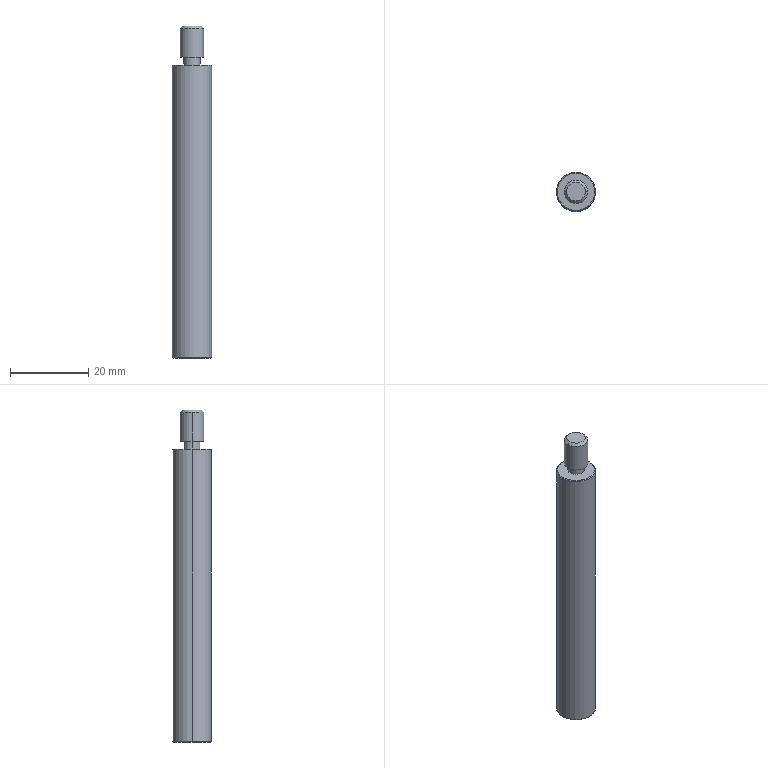Component | SolidWorks | Q1-A12-S21-Q1A.SLDASQ-1_Q1-VAFD10-75-F10-Q6-N5-1 | 1 solid | 22 faces | box 10 x 10 x 85 mm | volume 5928 mm3 | cone 10 | cylinder 8 | plane 4 | commonest cylinder face diameters 4.134 x2 6 x2 4.2 x2 10 x2
build123d program:
from build123d import *

# Parameters (mm, degrees)
SKETCH2_W = 2
SKETCH2_H = 10


with BuildPart() as part:
    # Sketch1 → Revolve1 (revolve)
    with BuildSketch(Plane.XY, mode=Mode.PRIVATE) as revolve1_sk:
        Polygon((-10, 0), (-10, 2.386), (-9.386, 3), (0, 3), (0, 4.8), (0.2, 5), (74.8, 5), (75, 4.8), (75, 0), align=None)
    revolve(revolve1_sk.sketch.rotate(Axis((75, 0, 0), (-1, 0, 0)), 270), axis=Axis((75, 0, 0), (-1, 0, 0)))

    # Sketch2 → Cut-Revolve1 (revolve, cut)
    with BuildSketch(Plane.XY, mode=Mode.PRIVATE) as cut_revolve1_sk:
        with Locations((-1, 7.1)):
            Rectangle(SKETCH2_W, SKETCH2_H)
    revolve(cut_revolve1_sk.sketch.rotate(Axis((85, 0, 0), (-1, 0, 0)), 270), axis=Axis((85, 0, 0), (-1, 0, 0)), mode=Mode.SUBTRACT)

    # Sketch3 → Cut-Revolve2 (revolve, cut)
    with BuildSketch(Plane.XY, mode=Mode.PRIVATE) as cut_revolve2_sk:
        Polygon((58.5, 0), (59.693, 2.067), (74.567, 2.067), (75, 2.5), (75, 0), align=None)
    revolve(cut_revolve2_sk.sketch.rotate(Axis((75, 0, 0), (-1, 0, 0)), 270), axis=Axis((75, 0, 0), (-1, 0, 0)), mode=Mode.SUBTRACT)


solid = part.part

# Placed as in the assembly
solid = solid.moved(Location((24.749, 24.749, -162.5), (0, 90, 0)))
STEP:
#1=COLOUR_RGB('',0.7922,0.8196,0.9333);
#2=FILL_AREA_STYLE_COLOUR('',#1);
#3=FILL_AREA_STYLE('',(#2));
#4=SURFACE_STYLE_FILL_AREA(#3);
#5=SURFACE_SIDE_STYLE('',(#4));
#6=SURFACE_STYLE_USAGE(.BOTH.,#5);
#7=PRESENTATION_STYLE_ASSIGNMENT((#6));
#8=CARTESIAN_POINT('',(0.9744,0.9744,-8.701));
#9=VERTEX_POINT('',#8);
#10=CARTESIAN_POINT('',(0.893,0.9744,-8.748));
#11=VERTEX_POINT('',#10);
#12=CARTESIAN_POINT('',(0.893,0.9744,-8.748));
#13=DIRECTION('',(-0.866,0.,-0.5));
#14=VECTOR('',#13,39.37);
#15=LINE('',#12,#14);
#16=EDGE_CURVE('',#9,#11,#15,.T.);
#17=ORIENTED_EDGE('',*,*,#16,.F.);
#18=CARTESIAN_POINT('',(1.056,0.9744,-8.748));
#19=VERTEX_POINT('',#18);
#20=CARTESIAN_POINT('',(1.056,0.9744,-8.748));
#21=DIRECTION('',(0.866,0.,-0.5));
#22=VECTOR('',#21,39.37);
#23=LINE('',#20,#22);
#24=EDGE_CURVE('',#9,#19,#23,.T.);
#25=ORIENTED_EDGE('',*,*,#24,.T.);
#26=CARTESIAN_POINT('',(0.9744,0.9744,-8.748));
#27=DIRECTION('',(0.,-0.,1.));
#28=DIRECTION('',(1.,0.,0.));
#29=AXIS2_PLACEMENT_3D('',#26,#27,#28);
#30=CIRCLE('',#29,0.08138);
#31=EDGE_CURVE('',#11,#19,#30,.T.);
#32=ORIENTED_EDGE('',*,*,#31,.F.);
#33=EDGE_LOOP('',(#17,#25,#32));
#34=FACE_OUTER_BOUND('',#33,.T.);
#35=CARTESIAN_POINT('',(0.9744,0.9744,-8.748));
#36=DIRECTION('',(-0.,0.,-1.));
#37=DIRECTION('',(-1.,0.,0.));
#38=AXIS2_PLACEMENT_3D('',#35,#36,#37);
#39=CONICAL_SURFACE('',#38,0.08138,1.047);
#40=ADVANCED_FACE('',(#34),#39,.F.);
#41=CARTESIAN_POINT('',(0.893,0.9744,-9.333));
#42=VERTEX_POINT('',#41);
#43=CARTESIAN_POINT('',(1.056,0.9744,-9.333));
#44=VERTEX_POINT('',#43);
#45=CARTESIAN_POINT('',(0.9744,0.9744,-9.333));
#46=DIRECTION('',(0.,-0.,1.));
#47=DIRECTION('',(1.,0.,0.));
#48=AXIS2_PLACEMENT_3D('',#45,#46,#47);
#49=CIRCLE('',#48,0.08138);
#50=EDGE_CURVE('',#42,#44,#49,.T.);
#51=ORIENTED_EDGE('',*,*,#50,.F.);
#52=CARTESIAN_POINT('',(0.893,0.9744,-9.35));
#53=DIRECTION('',(0.,-0.,1.));
#54=VECTOR('',#53,39.37);
#55=LINE('',#52,#54);
#56=EDGE_CURVE('',#42,#11,#55,.T.);
#57=ORIENTED_EDGE('',*,*,#56,.T.);
#58=ORIENTED_EDGE('',*,*,#31,.T.);
#59=CARTESIAN_POINT('',(1.056,0.9744,-9.35));
#60=DIRECTION('',(0.,-0.,1.));
#61=VECTOR('',#60,39.37);
#62=LINE('',#59,#61);
#63=EDGE_CURVE('',#44,#19,#62,.T.);
#64=ORIENTED_EDGE('',*,*,#63,.F.);
#65=EDGE_LOOP('',(#51,#57,#58,#64));
#66=FACE_OUTER_BOUND('',#65,.T.);
#67=CARTESIAN_POINT('',(0.9744,0.9744,-9.35));
#68=DIRECTION('',(0.,-0.,1.));
#69=DIRECTION('',(1.,0.,0.));
#70=AXIS2_PLACEMENT_3D('',#67,#68,#69);
#71=CYLINDRICAL_SURFACE('',#70,0.08138);
#72=ADVANCED_FACE('',(#66),#71,.F.);
#73=ORIENTED_EDGE('',*,*,#50,.T.);
#74=CARTESIAN_POINT('',(1.073,0.9744,-9.35));
#75=VERTEX_POINT('',#74);
#76=CARTESIAN_POINT('',(1.073,0.9744,-9.35));
#77=DIRECTION('',(0.7071,0.,-0.7071));
#78=VECTOR('',#77,39.37);
#79=LINE('',#76,#78);
#80=EDGE_CURVE('',#44,#75,#79,.T.);
#81=ORIENTED_EDGE('',*,*,#80,.T.);
#82=CARTESIAN_POINT('',(0.8759,0.9744,-9.35));
#83=VERTEX_POINT('',#82);
#84=CARTESIAN_POINT('',(0.9744,0.9744,-9.35));
#85=DIRECTION('',(0.,-0.,1.));
#86=DIRECTION('',(1.,0.,0.));
#87=AXIS2_PLACEMENT_3D('',#84,#85,#86);
#88=CIRCLE('',#87,0.09843);
#89=EDGE_CURVE('',#83,#75,#88,.T.);
#90=ORIENTED_EDGE('',*,*,#89,.F.);
#91=CARTESIAN_POINT('',(0.8759,0.9744,-9.35));
#92=DIRECTION('',(-0.7071,0.,-0.7071));
#93=VECTOR('',#92,39.37);
#94=LINE('',#91,#93);
#95=EDGE_CURVE('',#42,#83,#94,.T.);
#96=ORIENTED_EDGE('',*,*,#95,.F.);
#97=EDGE_LOOP('',(#73,#81,#90,#96));
#98=FACE_OUTER_BOUND('',#97,.T.);
#99=CARTESIAN_POINT('',(0.9744,0.9744,-9.35));
#100=DIRECTION('',(-0.,0.,-1.));
#101=DIRECTION('',(-1.,0.,0.));
#102=AXIS2_PLACEMENT_3D('',#99,#100,#101);
#103=CONICAL_SURFACE('',#102,0.09843,0.7854);
#104=ADVANCED_FACE('',(#98),#103,.F.);
#105=CARTESIAN_POINT('',(0.8562,0.9744,-6.319));
#106=VERTEX_POINT('',#105);
#107=CARTESIAN_POINT('',(1.092,0.9744,-6.319));
#108=VERTEX_POINT('',#107);
#109=CARTESIAN_POINT('',(0.9744,0.9744,-6.319));
#110=DIRECTION('',(-0.,0.,-1.));
#111=DIRECTION('',(-1.,0.,0.));
#112=AXIS2_PLACEMENT_3D('',#109,#110,#111);
#113=CIRCLE('',#112,0.1181);
#114=EDGE_CURVE('',#106,#108,#113,.T.);
#115=ORIENTED_EDGE('',*,*,#114,.F.);
#116=CARTESIAN_POINT('',(0.8562,0.9744,-6.028));
#117=VERTEX_POINT('',#116);
#118=CARTESIAN_POINT('',(0.8562,0.9744,-9.35));
#119=DIRECTION('',(0.,-0.,1.));
#120=VECTOR('',#119,39.37);
#121=LINE('',#118,#120);
#122=EDGE_CURVE('',#106,#117,#121,.T.);
#123=ORIENTED_EDGE('',*,*,#122,.T.);
#124=CARTESIAN_POINT('',(1.092,0.9744,-6.028));
#125=VERTEX_POINT('',#124);
#126=CARTESIAN_POINT('',(0.9744,0.9744,-6.028));
#127=DIRECTION('',(0.,-0.,1.));
#128=DIRECTION('',(1.,0.,0.));
#129=AXIS2_PLACEMENT_3D('',#126,#127,#128);
#130=CIRCLE('',#129,0.1181);
#131=EDGE_CURVE('',#125,#117,#130,.T.);
#132=ORIENTED_EDGE('',*,*,#131,.F.);
#133=CARTESIAN_POINT('',(1.092,0.9744,-9.35));
#134=DIRECTION('',(0.,-0.,1.));
#135=VECTOR('',#134,39.37);
#136=LINE('',#133,#135);
#137=EDGE_CURVE('',#108,#125,#136,.T.);
#138=ORIENTED_EDGE('',*,*,#137,.F.);
#139=EDGE_LOOP('',(#115,#123,#132,#138));
#140=FACE_OUTER_BOUND('',#139,.T.);
#141=CARTESIAN_POINT('',(0.9744,0.9744,-9.35));
#142=DIRECTION('',(0.,-0.,1.));
#143=DIRECTION('',(1.,0.,0.));
#144=AXIS2_PLACEMENT_3D('',#141,#142,#143);
#145=CYLINDRICAL_SURFACE('',#144,0.1181);
#146=ADVANCED_FACE('',(#140),#145,.T.);
#147=CARTESIAN_POINT('',(1.068,0.9744,-6.004));
#148=VERTEX_POINT('',#147);
#149=CARTESIAN_POINT('',(0.8804,0.9744,-6.004));
#150=VERTEX_POINT('',#149);
#151=CARTESIAN_POINT('',(0.9744,0.9744,-6.004));
#152=DIRECTION('',(0.,-0.,1.));
#153=DIRECTION('',(1.,0.,0.));
#154=AXIS2_PLACEMENT_3D('',#151,#152,#153);
#155=CIRCLE('',#154,0.09396);
#156=EDGE_CURVE('',#148,#150,#155,.T.);
#157=ORIENTED_EDGE('',*,*,#156,.F.);
#158=CARTESIAN_POINT('',(1.092,0.9744,-6.028));
#159=DIRECTION('',(0.7071,0.,-0.7071));
#160=VECTOR('',#159,39.37);
#161=LINE('',#158,#160);
#162=EDGE_CURVE('',#148,#125,#161,.T.);
#163=ORIENTED_EDGE('',*,*,#162,.T.);
#164=ORIENTED_EDGE('',*,*,#131,.T.);
#165=CARTESIAN_POINT('',(0.8562,0.9744,-6.028));
#166=DIRECTION('',(-0.7071,0.,-0.7071));
#167=VECTOR('',#166,39.37);
#168=LINE('',#165,#167);
#169=EDGE_CURVE('',#150,#117,#168,.T.);
#170=ORIENTED_EDGE('',*,*,#169,.F.);
#171=EDGE_LOOP('',(#157,#163,#164,#170));
#172=FACE_OUTER_BOUND('',#171,.T.);
#173=CARTESIAN_POINT('',(0.9744,0.9744,-6.028));
#174=DIRECTION('',(-0.,0.,-1.));
#175=DIRECTION('',(-1.,0.,0.));
#176=AXIS2_PLACEMENT_3D('',#173,#174,#175);
#177=CONICAL_SURFACE('',#176,0.1181,0.7854);
#178=ADVANCED_FACE('',(#172),#177,.T.);
#179=CARTESIAN_POINT('',(1.057,0.9744,-6.398));
#180=VERTEX_POINT('',#179);
#181=CARTESIAN_POINT('',(0.8917,0.9744,-6.398));
#182=VERTEX_POINT('',#181);
#183=CARTESIAN_POINT('',(0.9744,0.9744,-6.398));
#184=DIRECTION('',(0.,-0.,1.));
#185=DIRECTION('',(1.,0.,0.));
#186=AXIS2_PLACEMENT_3D('',#183,#184,#185);
#187=CIRCLE('',#186,0.08268);
#188=EDGE_CURVE('',#180,#182,#187,.T.);
#189=ORIENTED_EDGE('',*,*,#188,.T.);
#190=CARTESIAN_POINT('',(0.8917,0.9744,-6.319));
#191=VERTEX_POINT('',#190);
#192=CARTESIAN_POINT('',(0.8917,0.9744,-9.744));
#193=DIRECTION('',(0.,-0.,1.));
#194=VECTOR('',#193,39.37);
#195=LINE('',#192,#194);
#196=EDGE_CURVE('',#182,#191,#195,.T.);
#197=ORIENTED_EDGE('',*,*,#196,.T.);
#198=CARTESIAN_POINT('',(1.057,0.9744,-6.319));
#199=VERTEX_POINT('',#198);
#200=CARTESIAN_POINT('',(0.9744,0.9744,-6.319));
#201=DIRECTION('',(0.,-0.,1.));
#202=DIRECTION('',(1.,0.,0.));
#203=AXIS2_PLACEMENT_3D('',#200,#201,#202);
#204=CIRCLE('',#203,0.08268);
#205=EDGE_CURVE('',#199,#191,#204,.T.);
#206=ORIENTED_EDGE('',*,*,#205,.F.);
#207=CARTESIAN_POINT('',(1.057,0.9744,-9.744));
#208=DIRECTION('',(0.,-0.,1.));
#209=VECTOR('',#208,39.37);
#210=LINE('',#207,#209);
#211=EDGE_CURVE('',#180,#199,#210,.T.);
#212=ORIENTED_EDGE('',*,*,#211,.F.);
#213=EDGE_LOOP('',(#189,#197,#206,#212));
#214=FACE_OUTER_BOUND('',#213,.T.);
#215=CARTESIAN_POINT('',(0.9744,0.9744,-9.744));
#216=DIRECTION('',(0.,-0.,1.));
#217=DIRECTION('',(1.,0.,0.));
#218=AXIS2_PLACEMENT_3D('',#215,#216,#217);
#219=CYLINDRICAL_SURFACE('',#218,0.08268);
#220=ADVANCED_FACE('',(#214),#219,.T.);
#221=CARTESIAN_POINT('',(1.163,0.9744,-9.35));
#222=VERTEX_POINT('',#221);
#223=CARTESIAN_POINT('',(0.7854,0.9744,-9.35));
#224=VERTEX_POINT('',#223);
#225=CARTESIAN_POINT('',(0.9744,0.9744,-9.35));
#226=DIRECTION('',(0.,-0.,1.));
#227=DIRECTION('',(1.,0.,0.));
#228=AXIS2_PLACEMENT_3D('',#225,#226,#227);
#229=CIRCLE('',#228,0.189);
#230=EDGE_CURVE('',#222,#224,#229,.T.);
#231=ORIENTED_EDGE('',*,*,#230,.T.);
#232=CARTESIAN_POINT('',(0.7775,0.9744,-9.343));
#233=VERTEX_POINT('',#232);
#234=CARTESIAN_POINT('',(0.7854,0.9744,-9.35));
#235=DIRECTION('',(-0.7071,0.,0.7071));
#236=VECTOR('',#235,39.37);
#237=LINE('',#234,#236);
#238=EDGE_CURVE('',#224,#233,#237,.T.);
#239=ORIENTED_EDGE('',*,*,#238,.T.);
#240=CARTESIAN_POINT('',(1.171,0.9744,-9.343));
#241=VERTEX_POINT('',#240);
#242=CARTESIAN_POINT('',(0.9744,0.9744,-9.343));
#243=DIRECTION('',(0.,-0.,1.));
#244=DIRECTION('',(1.,0.,0.));
#245=AXIS2_PLACEMENT_3D('',#242,#243,#244);
#246=CIRCLE('',#245,0.1969);
#247=EDGE_CURVE('',#241,#233,#246,.T.);
#248=ORIENTED_EDGE('',*,*,#247,.F.);
#249=CARTESIAN_POINT('',(1.163,0.9744,-9.35));
#250=DIRECTION('',(0.7071,-0.,0.7071));
#251=VECTOR('',#250,39.37);
#252=LINE('',#249,#251);
#253=EDGE_CURVE('',#222,#241,#252,.T.);
#254=ORIENTED_EDGE('',*,*,#253,.F.);
#255=EDGE_LOOP('',(#231,#239,#248,#254));
#256=FACE_OUTER_BOUND('',#255,.T.);
#257=CARTESIAN_POINT('',(0.9744,0.9744,-9.35));
#258=DIRECTION('',(0.,-0.,1.));
#259=DIRECTION('',(1.,0.,0.));
#260=AXIS2_PLACEMENT_3D('',#257,#258,#259);
#261=CONICAL_SURFACE('',#260,0.189,0.7854);
#262=ADVANCED_FACE('',(#256),#261,.T.);
#263=ORIENTED_EDGE('',*,*,#247,.T.);
#264=CARTESIAN_POINT('',(0.7775,0.9744,-6.406));
#265=VERTEX_POINT('',#264);
#266=CARTESIAN_POINT('',(0.7775,0.9744,-9.35));
#267=DIRECTION('',(0.,-0.,1.));
#268=VECTOR('',#267,39.37);
#269=LINE('',#266,#268);
#270=EDGE_CURVE('',#233,#265,#269,.T.);
#271=ORIENTED_EDGE('',*,*,#270,.T.);
#272=CARTESIAN_POINT('',(1.171,0.9744,-6.406));
#273=VERTEX_POINT('',#272);
#274=CARTESIAN_POINT('',(0.9744,0.9744,-6.406));
#275=DIRECTION('',(0.,-0.,1.));
#276=DIRECTION('',(1.,0.,0.));
#277=AXIS2_PLACEMENT_3D('',#274,#275,#276);
#278=CIRCLE('',#277,0.1969);
#279=EDGE_CURVE('',#273,#265,#278,.T.);
#280=ORIENTED_EDGE('',*,*,#279,.F.);
#281=CARTESIAN_POINT('',(1.171,0.9744,-9.35));
#282=DIRECTION('',(0.,-0.,1.));
#283=VECTOR('',#282,39.37);
#284=LINE('',#281,#283);
#285=EDGE_CURVE('',#241,#273,#284,.T.);
#286=ORIENTED_EDGE('',*,*,#285,.F.);
#287=EDGE_LOOP('',(#263,#271,#280,#286));
#288=FACE_OUTER_BOUND('',#287,.T.);
#289=CARTESIAN_POINT('',(0.9744,0.9744,-9.35));
#290=DIRECTION('',(0.,-0.,1.));
#291=DIRECTION('',(1.,0.,0.));
#292=AXIS2_PLACEMENT_3D('',#289,#290,#291);
#293=CYLINDRICAL_SURFACE('',#292,0.1969);
#294=ADVANCED_FACE('',(#288),#293,.T.);
#295=CARTESIAN_POINT('',(1.163,0.9744,-6.398));
#296=VERTEX_POINT('',#295);
#297=CARTESIAN_POINT('',(0.7854,0.9744,-6.398));
#298=VERTEX_POINT('',#297);
#299=CARTESIAN_POINT('',(0.9744,0.9744,-6.398));
#300=DIRECTION('',(0.,-0.,1.));
#301=DIRECTION('',(1.,0.,0.));
#302=AXIS2_PLACEMENT_3D('',#299,#300,#301);
#303=CIRCLE('',#302,0.189);
#304=EDGE_CURVE('',#296,#298,#303,.T.);
#305=ORIENTED_EDGE('',*,*,#304,.F.);
#306=CARTESIAN_POINT('',(1.171,0.9744,-6.406));
#307=DIRECTION('',(0.7071,0.,-0.7071));
#308=VECTOR('',#307,39.37);
#309=LINE('',#306,#308);
#310=EDGE_CURVE('',#296,#273,#309,.T.);
#311=ORIENTED_EDGE('',*,*,#310,.T.);
#312=ORIENTED_EDGE('',*,*,#279,.T.);
#313=CARTESIAN_POINT('',(0.7775,0.9744,-6.406));
#314=DIRECTION('',(-0.7071,0.,-0.7071));
#315=VECTOR('',#314,39.37);
#316=LINE('',#313,#315);
#317=EDGE_CURVE('',#298,#265,#316,.T.);
#318=ORIENTED_EDGE('',*,*,#317,.F.);
#319=EDGE_LOOP('',(#305,#311,#312,#318));
#320=FACE_OUTER_BOUND('',#319,.T.);
#321=CARTESIAN_POINT('',(0.9744,0.9744,-6.406));
#322=DIRECTION('',(-0.,0.,-1.));
#323=DIRECTION('',(-1.,0.,0.));
#324=AXIS2_PLACEMENT_3D('',#321,#322,#323);
#325=CONICAL_SURFACE('',#324,0.1969,0.7854);
#326=ADVANCED_FACE('',(#320),#325,.T.);
#327=CARTESIAN_POINT('',(0.9744,0.9744,-6.398));
#328=DIRECTION('',(0.,-0.,1.));
#329=DIRECTION('',(1.,0.,0.));
#330=AXIS2_PLACEMENT_3D('',#327,#328,#329);
#331=CIRCLE('',#330,0.189);
#332=EDGE_CURVE('',#298,#296,#331,.T.);
#333=ORIENTED_EDGE('',*,*,#332,.T.);
#334=ORIENTED_EDGE('',*,*,#304,.T.);
#335=EDGE_LOOP('',(#333,#334));
#336=FACE_OUTER_BOUND('',#335,.T.);
#337=ORIENTED_EDGE('',*,*,#188,.F.);
#338=CARTESIAN_POINT('',(0.9744,0.9744,-6.398));
#339=DIRECTION('',(0.,-0.,1.));
#340=DIRECTION('',(1.,0.,0.));
#341=AXIS2_PLACEMENT_3D('',#338,#339,#340);
#342=CIRCLE('',#341,0.08268);
#343=EDGE_CURVE('',#182,#180,#342,.T.);
#344=ORIENTED_EDGE('',*,*,#343,.F.);
#345=EDGE_LOOP('',(#337,#344));
#346=FACE_BOUND('',#345,.T.);
#347=CARTESIAN_POINT('',(0.9744,1.092,-6.398));
#348=DIRECTION('',(0.,0.,-1.));
#349=DIRECTION('',(-1.,0.,-0.));
#350=AXIS2_PLACEMENT_3D('',#347,#348,#349);
#351=PLANE('',#350);
#352=ADVANCED_FACE('',(#336,#346),#351,.F.);
#353=ORIENTED_EDGE('',*,*,#310,.F.);
#354=ORIENTED_EDGE('',*,*,#332,.F.);
#355=ORIENTED_EDGE('',*,*,#317,.T.);
#356=CARTESIAN_POINT('',(0.9744,0.9744,-6.406));
#357=DIRECTION('',(0.,-0.,1.));
#358=DIRECTION('',(1.,0.,0.));
#359=AXIS2_PLACEMENT_3D('',#356,#357,#358);
#360=CIRCLE('',#359,0.1969);
#361=EDGE_CURVE('',#265,#273,#360,.T.);
#362=ORIENTED_EDGE('',*,*,#361,.T.);
#363=EDGE_LOOP('',(#353,#354,#355,#362));
#364=FACE_OUTER_BOUND('',#363,.T.);
#365=CARTESIAN_POINT('',(0.9744,0.9744,-6.406));
#366=DIRECTION('',(-0.,0.,-1.));
#367=DIRECTION('',(-1.,0.,0.));
#368=AXIS2_PLACEMENT_3D('',#365,#366,#367);
#369=CONICAL_SURFACE('',#368,0.1969,0.7854);
#370=ADVANCED_FACE('',(#364),#369,.T.);
#371=ORIENTED_EDGE('',*,*,#270,.F.);
#372=CARTESIAN_POINT('',(0.9744,0.9744,-9.343));
#373=DIRECTION('',(0.,-0.,1.));
#374=DIRECTION('',(1.,0.,0.));
#375=AXIS2_PLACEMENT_3D('',#372,#373,#374);
#376=CIRCLE('',#375,0.1969);
#377=EDGE_CURVE('',#233,#241,#376,.T.);
#378=ORIENTED_EDGE('',*,*,#377,.T.);
#379=ORIENTED_EDGE('',*,*,#285,.T.);
#380=ORIENTED_EDGE('',*,*,#361,.F.);
#381=EDGE_LOOP('',(#371,#378,#379,#380));
#382=FACE_OUTER_BOUND('',#381,.T.);
#383=CARTESIAN_POINT('',(0.9744,0.9744,-9.35));
#384=DIRECTION('',(0.,-0.,1.));
#385=DIRECTION('',(1.,0.,0.));
#386=AXIS2_PLACEMENT_3D('',#383,#384,#385);
#387=CYLINDRICAL_SURFACE('',#386,0.1969);
#388=ADVANCED_FACE('',(#382),#387,.T.);
#389=ORIENTED_EDGE('',*,*,#238,.F.);
#390=CARTESIAN_POINT('',(0.9744,0.9744,-9.35));
#391=DIRECTION('',(0.,-0.,1.));
#392=DIRECTION('',(1.,0.,0.));
#393=AXIS2_PLACEMENT_3D('',#390,#391,#392);
#394=CIRCLE('',#393,0.189);
#395=EDGE_CURVE('',#224,#222,#394,.T.);
#396=ORIENTED_EDGE('',*,*,#395,.T.);
#397=ORIENTED_EDGE('',*,*,#253,.T.);
#398=ORIENTED_EDGE('',*,*,#377,.F.);
#399=EDGE_LOOP('',(#389,#396,#397,#398));
#400=FACE_OUTER_BOUND('',#399,.T.);
#401=CARTESIAN_POINT('',(0.9744,0.9744,-9.35));
#402=DIRECTION('',(0.,-0.,1.));
#403=DIRECTION('',(1.,0.,0.));
#404=AXIS2_PLACEMENT_3D('',#401,#402,#403);
#405=CONICAL_SURFACE('',#404,0.189,0.7854);
#406=ADVANCED_FACE('',(#400),#405,.T.);
#407=ORIENTED_EDGE('',*,*,#89,.T.);
#408=CARTESIAN_POINT('',(0.9744,0.9744,-9.35));
#409=DIRECTION('',(0.,-0.,1.));
#410=DIRECTION('',(1.,0.,0.));
#411=AXIS2_PLACEMENT_3D('',#408,#409,#410);
#412=CIRCLE('',#411,0.09843);
#413=EDGE_CURVE('',#75,#83,#412,.T.);
#414=ORIENTED_EDGE('',*,*,#413,.T.);
#415=EDGE_LOOP('',(#407,#414));
#416=FACE_BOUND('',#415,.T.);
#417=ORIENTED_EDGE('',*,*,#230,.F.);
#418=ORIENTED_EDGE('',*,*,#395,.F.);
#419=EDGE_LOOP('',(#417,#418));
#420=FACE_OUTER_BOUND('',#419,.T.);
#421=CARTESIAN_POINT('',(0.9744,1.163,-9.35));
#422=DIRECTION('',(-0.,-0.,1.));
#423=DIRECTION('',(1.,-0.,0.));
#424=AXIS2_PLACEMENT_3D('',#421,#422,#423);
#425=PLANE('',#424);
#426=ADVANCED_FACE('',(#416,#420),#425,.F.);
#427=ORIENTED_EDGE('',*,*,#205,.T.);
#428=CARTESIAN_POINT('',(0.9744,0.9744,-6.319));
#429=DIRECTION('',(0.,-0.,1.));
#430=DIRECTION('',(1.,0.,0.));
#431=AXIS2_PLACEMENT_3D('',#428,#429,#430);
#432=CIRCLE('',#431,0.08268);
#433=EDGE_CURVE('',#191,#199,#432,.T.);
#434=ORIENTED_EDGE('',*,*,#433,.T.);
#435=EDGE_LOOP('',(#427,#434));
#436=FACE_BOUND('',#435,.T.);
#437=CARTESIAN_POINT('',(0.9744,0.9744,-6.319));
#438=DIRECTION('',(-0.,0.,-1.));
#439=DIRECTION('',(-1.,0.,0.));
#440=AXIS2_PLACEMENT_3D('',#437,#438,#439);
#441=CIRCLE('',#440,0.1181);
#442=EDGE_CURVE('',#108,#106,#441,.T.);
#443=ORIENTED_EDGE('',*,*,#442,.T.);
#444=ORIENTED_EDGE('',*,*,#114,.T.);
#445=EDGE_LOOP('',(#443,#444));
#446=FACE_OUTER_BOUND('',#445,.T.);
#447=CARTESIAN_POINT('',(0.9744,1.451,-6.319));
#448=DIRECTION('',(0.,0.,-1.));
#449=DIRECTION('',(-1.,0.,-0.));
#450=AXIS2_PLACEMENT_3D('',#447,#448,#449);
#451=PLANE('',#450);
#452=ADVANCED_FACE('',(#436,#446),#451,.T.);
#453=ORIENTED_EDGE('',*,*,#196,.F.);
#454=ORIENTED_EDGE('',*,*,#343,.T.);
#455=ORIENTED_EDGE('',*,*,#211,.T.);
#456=ORIENTED_EDGE('',*,*,#433,.F.);
#457=EDGE_LOOP('',(#453,#454,#455,#456));
#458=FACE_OUTER_BOUND('',#457,.T.);
#459=CARTESIAN_POINT('',(0.9744,0.9744,-9.744));
#460=DIRECTION('',(0.,-0.,1.));
#461=DIRECTION('',(1.,0.,0.));
#462=AXIS2_PLACEMENT_3D('',#459,#460,#461);
#463=CYLINDRICAL_SURFACE('',#462,0.08268);
#464=ADVANCED_FACE('',(#458),#463,.T.);
#465=CARTESIAN_POINT('',(0.9744,0.9744,-6.004));
#466=DIRECTION('',(0.,-0.,1.));
#467=DIRECTION('',(1.,0.,0.));
#468=AXIS2_PLACEMENT_3D('',#465,#466,#467);
#469=CIRCLE('',#468,0.09396);
#470=EDGE_CURVE('',#150,#148,#469,.T.);
#471=ORIENTED_EDGE('',*,*,#470,.T.);
#472=ORIENTED_EDGE('',*,*,#156,.T.);
#473=EDGE_LOOP('',(#471,#472));
#474=FACE_OUTER_BOUND('',#473,.T.);
#475=CARTESIAN_POINT('',(0.9744,0.9744,-6.004));
#476=DIRECTION('',(0.,0.,-1.));
#477=DIRECTION('',(-1.,0.,-0.));
#478=AXIS2_PLACEMENT_3D('',#475,#476,#477);
#479=PLANE('',#478);
#480=ADVANCED_FACE('',(#474),#479,.F.);
#481=ORIENTED_EDGE('',*,*,#162,.F.);
#482=ORIENTED_EDGE('',*,*,#470,.F.);
#483=ORIENTED_EDGE('',*,*,#169,.T.);
#484=CARTESIAN_POINT('',(0.9744,0.9744,-6.028));
#485=DIRECTION('',(0.,-0.,1.));
#486=DIRECTION('',(1.,0.,0.));
#487=AXIS2_PLACEMENT_3D('',#484,#485,#486);
#488=CIRCLE('',#487,0.1181);
#489=EDGE_CURVE('',#117,#125,#488,.T.);
#490=ORIENTED_EDGE('',*,*,#489,.T.);
#491=EDGE_LOOP('',(#481,#482,#483,#490));
#492=FACE_OUTER_BOUND('',#491,.T.);
#493=CARTESIAN_POINT('',(0.9744,0.9744,-6.028));
#494=DIRECTION('',(-0.,0.,-1.));
#495=DIRECTION('',(-1.,0.,0.));
#496=AXIS2_PLACEMENT_3D('',#493,#494,#495);
#497=CONICAL_SURFACE('',#496,0.1181,0.7854);
#498=ADVANCED_FACE('',(#492),#497,.T.);
#499=ORIENTED_EDGE('',*,*,#122,.F.);
#500=ORIENTED_EDGE('',*,*,#442,.F.);
#501=ORIENTED_EDGE('',*,*,#137,.T.);
#502=ORIENTED_EDGE('',*,*,#489,.F.);
#503=EDGE_LOOP('',(#499,#500,#501,#502));
#504=FACE_OUTER_BOUND('',#503,.T.);
#505=CARTESIAN_POINT('',(0.9744,0.9744,-9.35));
#506=DIRECTION('',(0.,-0.,1.));
#507=DIRECTION('',(1.,0.,0.));
#508=AXIS2_PLACEMENT_3D('',#505,#506,#507);
#509=CYLINDRICAL_SURFACE('',#508,0.1181);
#510=ADVANCED_FACE('',(#504),#509,.T.);
#511=ORIENTED_EDGE('',*,*,#80,.F.);
#512=CARTESIAN_POINT('',(0.9744,0.9744,-9.333));
#513=DIRECTION('',(0.,-0.,1.));
#514=DIRECTION('',(1.,0.,0.));
#515=AXIS2_PLACEMENT_3D('',#512,#513,#514);
#516=CIRCLE('',#515,0.08138);
#517=EDGE_CURVE('',#44,#42,#516,.T.);
#518=ORIENTED_EDGE('',*,*,#517,.T.);
#519=ORIENTED_EDGE('',*,*,#95,.T.);
#520=ORIENTED_EDGE('',*,*,#413,.F.);
#521=EDGE_LOOP('',(#511,#518,#519,#520));
#522=FACE_OUTER_BOUND('',#521,.T.);
#523=CARTESIAN_POINT('',(0.9744,0.9744,-9.35));
#524=DIRECTION('',(-0.,0.,-1.));
#525=DIRECTION('',(-1.,0.,0.));
#526=AXIS2_PLACEMENT_3D('',#523,#524,#525);
#527=CONICAL_SURFACE('',#526,0.09843,0.7854);
#528=ADVANCED_FACE('',(#522),#527,.F.);
#529=ORIENTED_EDGE('',*,*,#56,.F.);
#530=ORIENTED_EDGE('',*,*,#517,.F.);
#531=ORIENTED_EDGE('',*,*,#63,.T.);
#532=CARTESIAN_POINT('',(0.9744,0.9744,-8.748));
#533=DIRECTION('',(0.,-0.,1.));
#534=DIRECTION('',(1.,0.,0.));
#535=AXIS2_PLACEMENT_3D('',#532,#533,#534);
#536=CIRCLE('',#535,0.08138);
#537=EDGE_CURVE('',#19,#11,#536,.T.);
#538=ORIENTED_EDGE('',*,*,#537,.T.);
#539=EDGE_LOOP('',(#529,#530,#531,#538));
#540=FACE_OUTER_BOUND('',#539,.T.);
#541=CARTESIAN_POINT('',(0.9744,0.9744,-9.35));
#542=DIRECTION('',(0.,-0.,1.));
#543=DIRECTION('',(1.,0.,0.));
#544=AXIS2_PLACEMENT_3D('',#541,#542,#543);
#545=CYLINDRICAL_SURFACE('',#544,0.08138);
#546=ADVANCED_FACE('',(#540),#545,.F.);
#547=ORIENTED_EDGE('',*,*,#24,.F.);
#548=ORIENTED_EDGE('',*,*,#16,.T.);
#549=ORIENTED_EDGE('',*,*,#537,.F.);
#550=EDGE_LOOP('',(#547,#548,#549));
#551=FACE_OUTER_BOUND('',#550,.T.);
#552=CARTESIAN_POINT('',(0.9744,0.9744,-8.748));
#553=DIRECTION('',(-0.,0.,-1.));
#554=DIRECTION('',(-1.,0.,0.));
#555=AXIS2_PLACEMENT_3D('',#552,#553,#554);
#556=CONICAL_SURFACE('',#555,0.08138,1.047);
#557=ADVANCED_FACE('',(#551),#556,.F.);
#558=CLOSED_SHELL('',(#40,#72,#104,#146,#178,#220,#262,#294,#326,#352,#370,#388,#406,#426,#452,#464,#480,#498,#510,#528,#546,#557));
#559=MANIFOLD_SOLID_BREP('',#558);
#560=STYLED_ITEM('',(#7),#559);
#561=PRESENTATION_LAYER_ASSIGNMENT('','',(#560));
#562=(LENGTH_UNIT()NAMED_UNIT(*)SI_UNIT($,.METRE.));
#563=LENGTH_MEASURE_WITH_UNIT(LENGTH_MEASURE(0.0254),#562);
#564=DIMENSIONAL_EXPONENTS(1.,0.,0.,0.,0.,0.,0.);
#565=(CONVERSION_BASED_UNIT('',#563)LENGTH_UNIT()NAMED_UNIT(#564));
#566=UNCERTAINTY_MEASURE_WITH_UNIT(LENGTH_MEASURE(0.00001),#565,'','');
#567=(NAMED_UNIT(*)PLANE_ANGLE_UNIT()SI_UNIT($,.RADIAN.));
#568=(NAMED_UNIT(*)SI_UNIT($,.STERADIAN.)SOLID_ANGLE_UNIT());
#569=(GEOMETRIC_REPRESENTATION_CONTEXT(3)GLOBAL_UNCERTAINTY_ASSIGNED_CONTEXT((#566))GLOBAL_UNIT_ASSIGNED_CONTEXT((#565,#567,#568))REPRESENTATION_CONTEXT('',''));
#570=MECHANICAL_DESIGN_GEOMETRIC_PRESENTATION_REPRESENTATION('',(#560),#569);
#571=CARTESIAN_POINT('',(0.,0.,0.));
#572=DIRECTION('',(0.,0.,1.));
#573=DIRECTION('',(1.,0.,0.));
#574=AXIS2_PLACEMENT_3D('',#571,#572,#573);
#575=(LENGTH_UNIT()NAMED_UNIT(*)SI_UNIT($,.METRE.));
#576=LENGTH_MEASURE_WITH_UNIT(LENGTH_MEASURE(0.0254),#575);
#577=DIMENSIONAL_EXPONENTS(1.,0.,0.,0.,0.,0.,0.);
#578=(CONVERSION_BASED_UNIT('',#576)LENGTH_UNIT()NAMED_UNIT(#577));
#579=UNCERTAINTY_MEASURE_WITH_UNIT(LENGTH_MEASURE(0.00001),#578,'','');
#580=(NAMED_UNIT(*)PLANE_ANGLE_UNIT()SI_UNIT($,.RADIAN.));
#581=(NAMED_UNIT(*)SI_UNIT($,.STERADIAN.)SOLID_ANGLE_UNIT());
#582=(GEOMETRIC_REPRESENTATION_CONTEXT(3)GLOBAL_UNCERTAINTY_ASSIGNED_CONTEXT((#579))GLOBAL_UNIT_ASSIGNED_CONTEXT((#578,#580,#581))REPRESENTATION_CONTEXT('',''));
#583=ADVANCED_BREP_SHAPE_REPRESENTATION('',(#559,#574),#582);